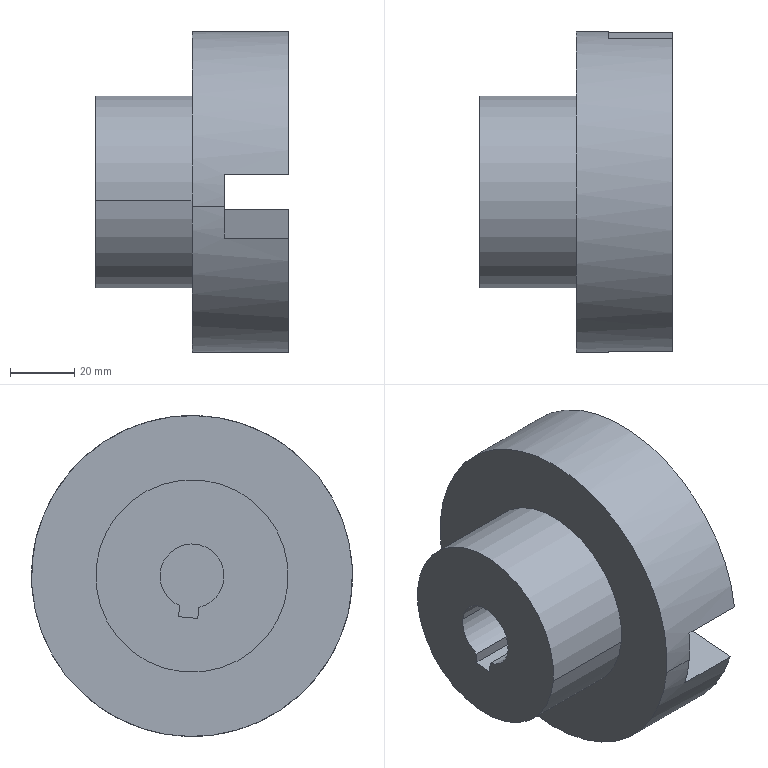Component | SolidWorks | CouplerAssembly-1_UpperCoupler-1 | 1 solid | 18 faces | box 60 x 100 x 100 mm | volume 274049 mm3 | plane 11 | cylinder 7 | commonest cylinder face diameters 20 x3 60 x2 100 x2
build123d program:
from build123d import *

# Parameters (mm, degrees)
SKETCH1_R           = 50
BOSS_EXTRUDE1_DEPTH = 30
CUT_EXTRUDE1_REACH  = 117.758
SKETCH3_W           = 20
SKETCH3_H           = 20
SKETCH4_R           = 30
BOSS_EXTRUDE2_DEPTH = 30
SKETCH5_R           = 10
CUT_EXTRUDE2_DEPTH  = 20
SKETCH6_W           = 6
SKETCH6_H           = 3.461
CUT_EXTRUDE3_DEPTH  = 20


with BuildPart() as part:
    # Sketch1 → Boss-Extrude1 (new body)
    with BuildSketch(Plane.XY):
        Circle(SKETCH1_R)
    extrude(amount=BOSS_EXTRUDE1_DEPTH)

    # Sketch3 → Cut-Extrude1 (cut, up to next)
    with BuildSketch(Plane(origin=(50, 0, 0), x_dir=(0, 0, -1), z_dir=(1, 0, 0)), mode=Mode.PRIVATE) as cut_extrude1_sk1:
        with Locations((-10, 0)):
            Rectangle(SKETCH3_W, SKETCH3_H)
    cut_extrude1_tool1 = extrude(cut_extrude1_sk1.sketch, amount=-CUT_EXTRUDE1_REACH, mode=Mode.PRIVATE) & part.part
    add(cut_extrude1_tool1.solids().sort_by_distance((50, 0, 10))[0], mode=Mode.SUBTRACT)

    # Sketch4 → Boss-Extrude2 (add)
    with BuildSketch(Plane.XY.offset(30)):
        Circle(SKETCH4_R)
    extrude(amount=BOSS_EXTRUDE2_DEPTH)

    # Sketch5 → Cut-Extrude2 (cut)
    with BuildSketch(Plane.XY.offset(60)):
        Circle(SKETCH5_R)
    extrude(amount=-CUT_EXTRUDE2_DEPTH, mode=Mode.SUBTRACT)

    # Sketch6 → Cut-Extrude3 (cut)
    with BuildSketch(Plane.XY.offset(60)):
        with Locations((0, -11.27)):
            Rectangle(SKETCH6_W, SKETCH6_H)
    extrude(amount=-CUT_EXTRUDE3_DEPTH, mode=Mode.SUBTRACT)


solid = part.part

# Placed as in the assembly
solid = solid.moved(Location((145.641, 70.663, 0), (95.194, -90, 0)))